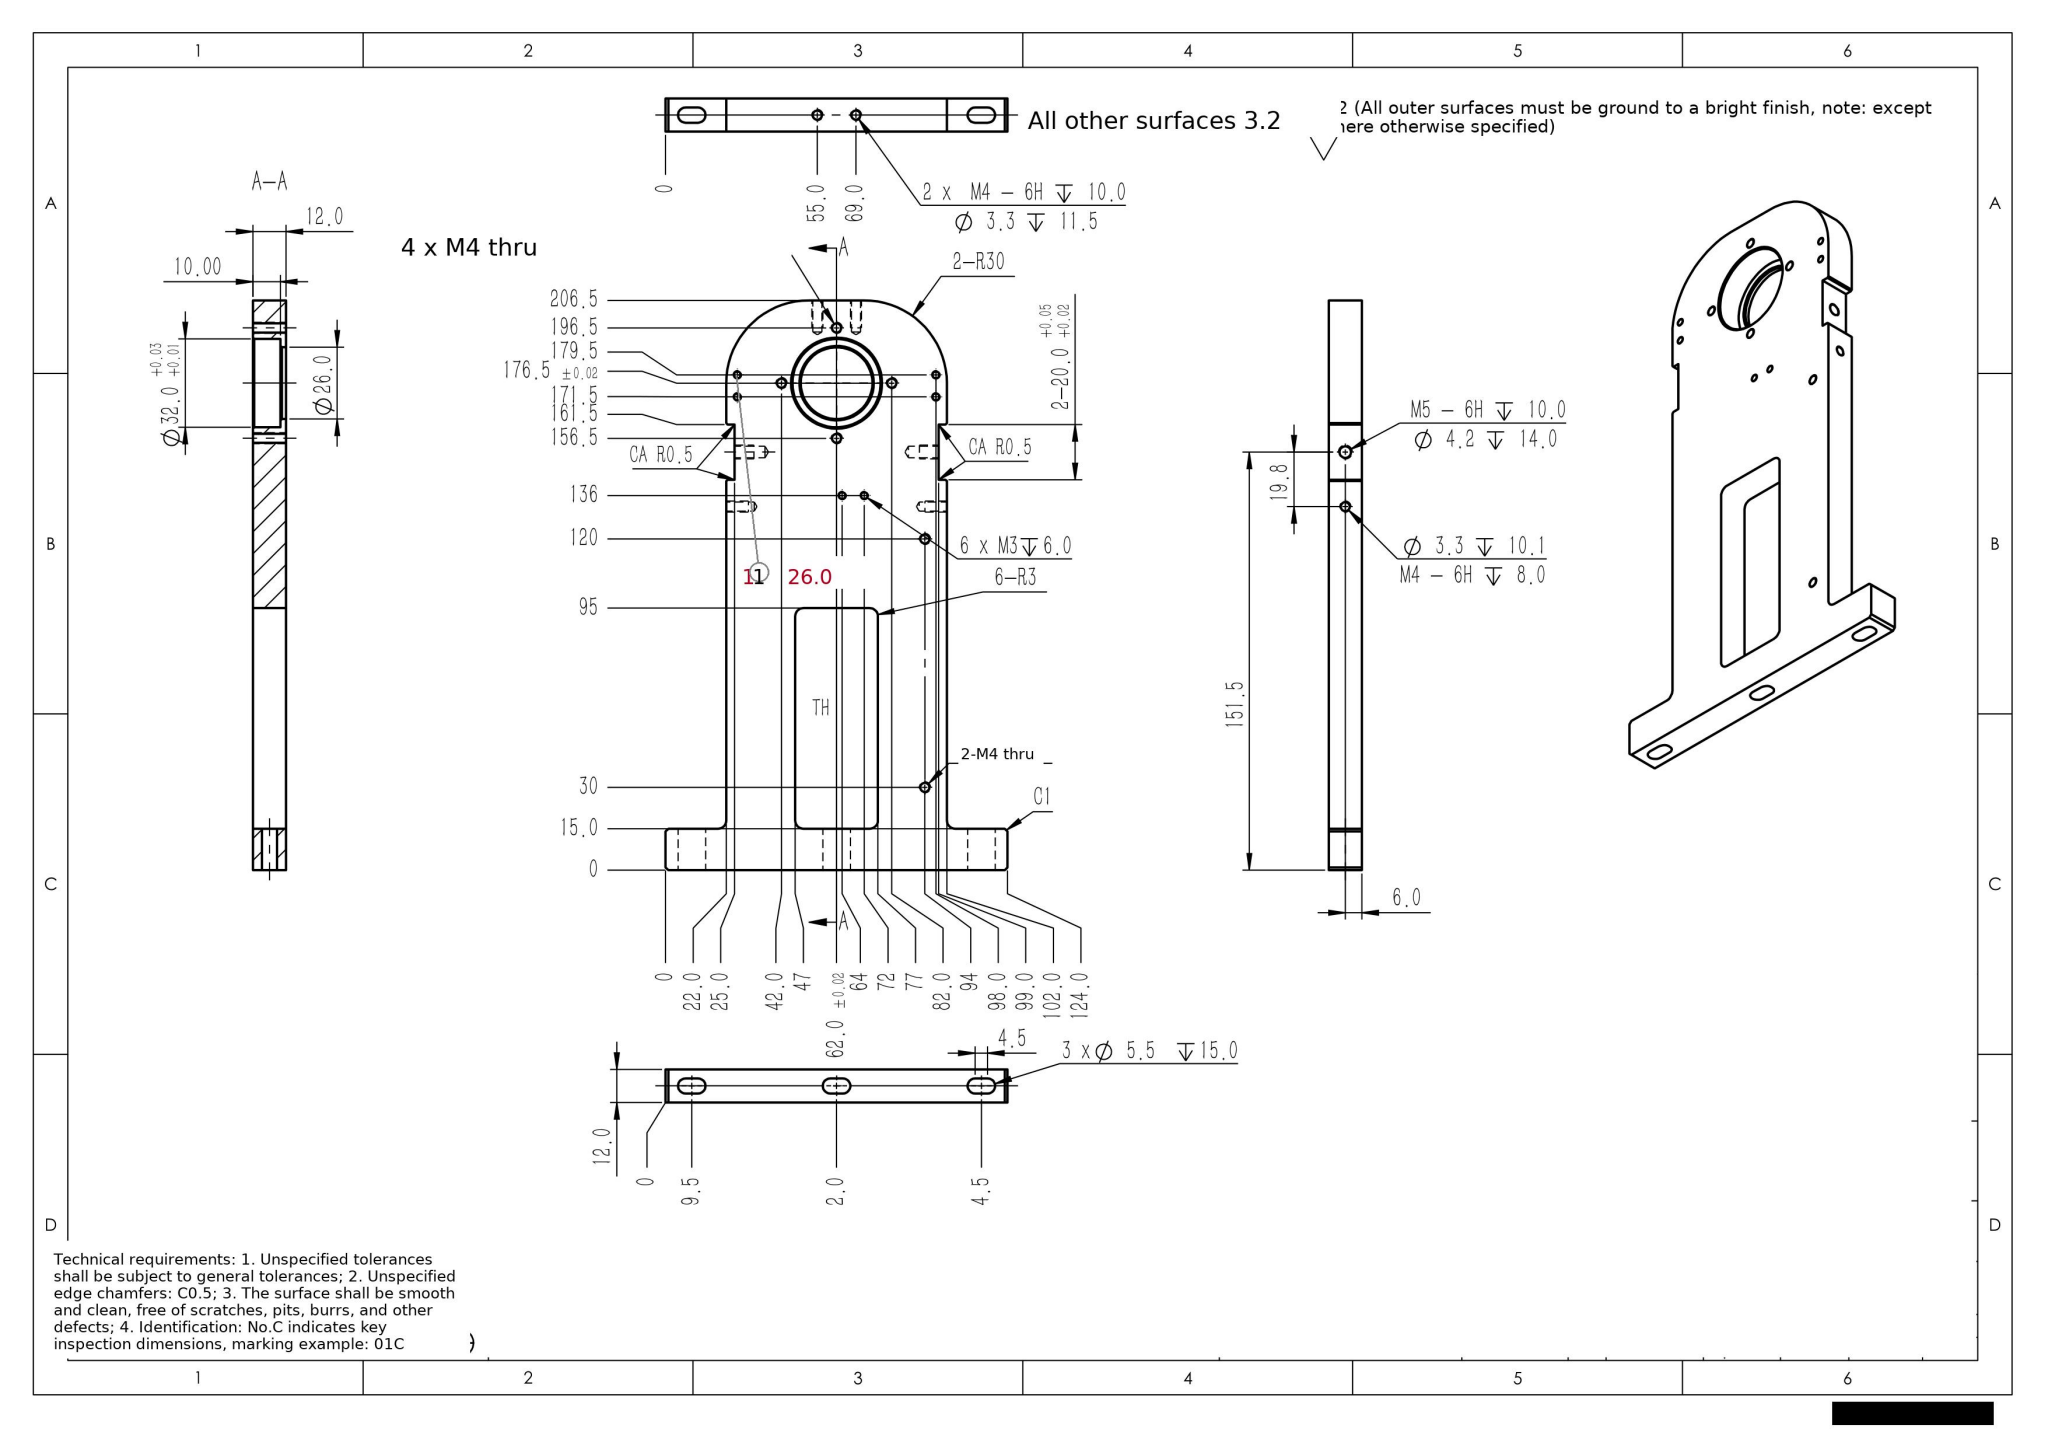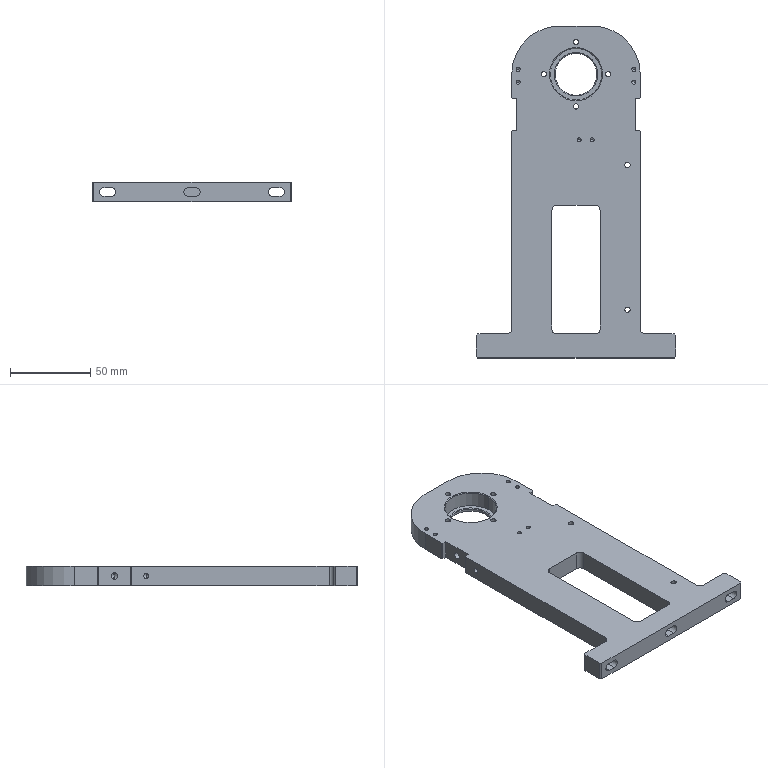Part | SolidWorks | mm | 1 solid | 119 faces | box 124 x 206.5 x 12 mm | volume 158513 mm3 | cylinder 54 | plane 37 | cone 28 | commonest cylinder face diameters 3.3 x20 2.5 x12 5.5 x6 6 x6 4.2 x4 26 x2 32 x2 60 x2